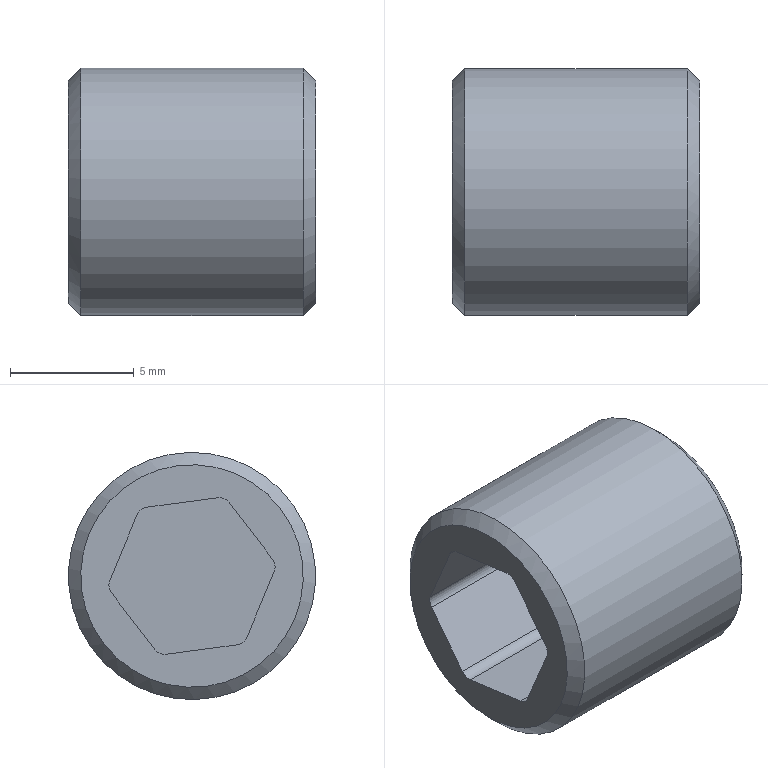Component | NX | SCREW_PLUG_2 | 1 solid | 18 faces | volume 622 mm3 | plane 9 | cylinder 7 | cone 2 | commonest cylinder face diameters 1 x6 10 x1